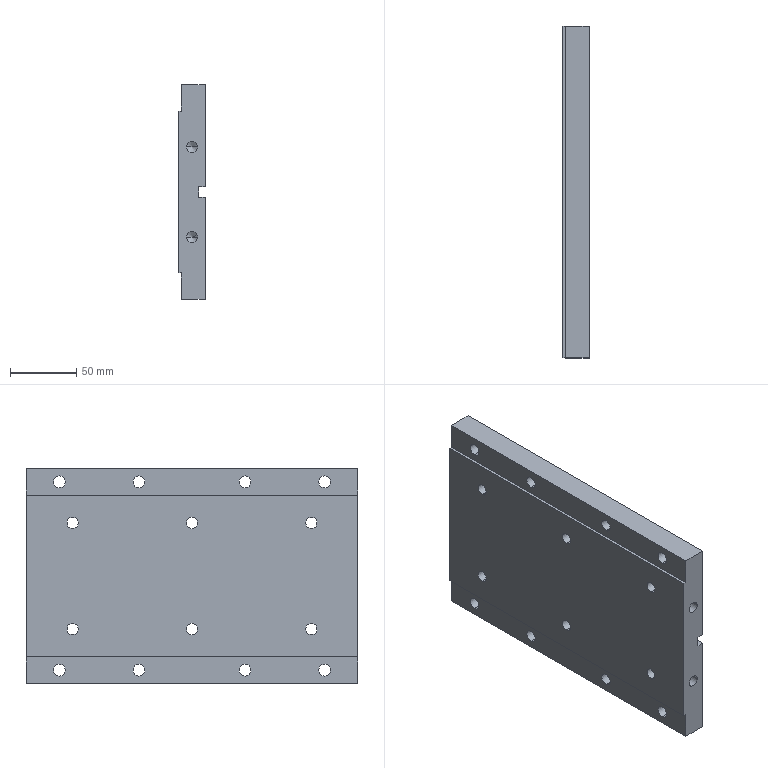Component | SolidWorks | F6-1 | 1 solid | 74 faces | box 20 x 250 x 162 mm | volume 753914 mm3 | cylinder 48 | plane 22 | cone 4 | commonest cylinder face diameters 8.5 x16 15 x16 9 x16
build123d program:
from build123d import *

# Parameters (mm, degrees)
SKETCH1_W                                       = 162
SKETCH1_H                                       = 250
BOSS_EXTRUDE1_DEPTH                             = 20
SKETCH2_W                                       = 8
SKETCH2_H                                       = 5
CUT_EXTRUDE1_DEPTH                              = 286.778
SKETCH3_W                                       = 20
SKETCH3_H                                       = 2
CUT_EXTRUDE2_DEPTH                              = 286.778
M8_HEX_SOCKET_HEAD_CAP_SCREW_CBORE1_D           = 9
M8_HEX_SOCKET_HEAD_CAP_SCREW_CBORE1_CBORE_D     = 15
M8_HEX_SOCKET_HEAD_CAP_SCREW_CBORE1_CBORE_DEPTH = 8
M10_TAPPED_HOLE1_D                              = 8.5
M10_TAPPED_HOLE1_DEPTH                          = 24.5
M10_TAPPED_HOLE1_TIP                            = 2.554
M10_TAPPED_HOLE2_D                              = 8.5
M10_TAPPED_HOLE2_DEPTH                          = 24.5
M10_TAPPED_HOLE2_TIP                            = 2.554


with BuildPart() as part:
    # Sketch1 → Boss-Extrude1 (new body)
    with BuildSketch(Plane.XY):
        with Locations((56, 588)):
            Rectangle(SKETCH1_W, SKETCH1_H)
    extrude(amount=BOSS_EXTRUDE1_DEPTH)

    # Sketch2 → Cut-Extrude1 (cut, through all)
    with BuildSketch(Plane.XZ.offset(-463)):
        with Locations((56, 17.5)):
            Rectangle(SKETCH2_W, SKETCH2_H)
    extrude(amount=-CUT_EXTRUDE1_DEPTH, mode=Mode.SUBTRACT)

    # Sketch3 → Cut-Extrude2 (cut, through all)
    with BuildSketch(Plane.XZ.offset(-463)):
        with Locations((-15, 1)):
            Rectangle(SKETCH3_W, SKETCH3_H)
        with Locations((127, 1)):
            Rectangle(SKETCH3_W, SKETCH3_H)
    extrude(amount=-CUT_EXTRUDE2_DEPTH, mode=Mode.SUBTRACT)

    # M8 Hex Socket Head Cap Screw CBORE1 (through all)
    with Locations(Plane.XY.offset(20)):
        with Locations((127, 688), (127, 628), (127, 548), (127, 488), (-15, 688), (-15, 628), (-15, 548), (-15, 488)):
            CounterBoreHole(M8_HEX_SOCKET_HEAD_CAP_SCREW_CBORE1_D / 2, M8_HEX_SOCKET_HEAD_CAP_SCREW_CBORE1_CBORE_D / 2, M8_HEX_SOCKET_HEAD_CAP_SCREW_CBORE1_CBORE_DEPTH)

    # M10 Tapped Hole1
    with Locations(Plane.XY.offset(20)):
        with Locations((16, 678), (96, 678), (96, 588), (96, 498), (16, 498), (16, 588)):
            Hole(M10_TAPPED_HOLE1_D / 2, depth=M10_TAPPED_HOLE1_DEPTH)
            with Locations((0, 0, -(M10_TAPPED_HOLE1_DEPTH + M10_TAPPED_HOLE1_TIP / 2))):  # 118° drill point
                Cone(0, M10_TAPPED_HOLE1_D / 2, M10_TAPPED_HOLE1_TIP, mode=Mode.SUBTRACT)

    # M10 Tapped Hole2
    with Locations(Plane.XZ.offset(-463)):
        with Locations((22, 10), (90, 10)):
            Hole(M10_TAPPED_HOLE2_D / 2, depth=M10_TAPPED_HOLE2_DEPTH)
            with Locations((0, 0, -(M10_TAPPED_HOLE2_DEPTH + M10_TAPPED_HOLE2_TIP / 2))):  # 118° drill point
                Cone(0, M10_TAPPED_HOLE2_D / 2, M10_TAPPED_HOLE2_TIP, mode=Mode.SUBTRACT)


solid = part.part

# Placed as in the assembly
solid = solid.moved(Location((76, -599.721, 0), (0, 90, 0)))